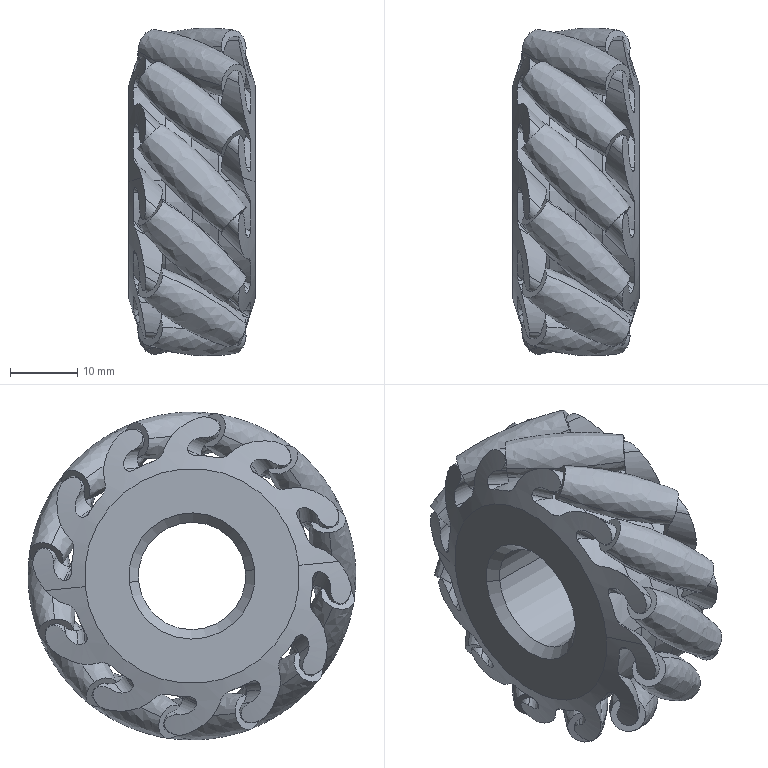Component | SolidWorks | MecanumWheel-1 | 1 solid | 252 faces | volume 22534 mm3 | cylinder 166 | plane 50 | spline 24 | cone 8 | torus 4 | commonest cylinder face diameters 4 x68 3.2 x36 16 x34 1.6 x24 36 x4